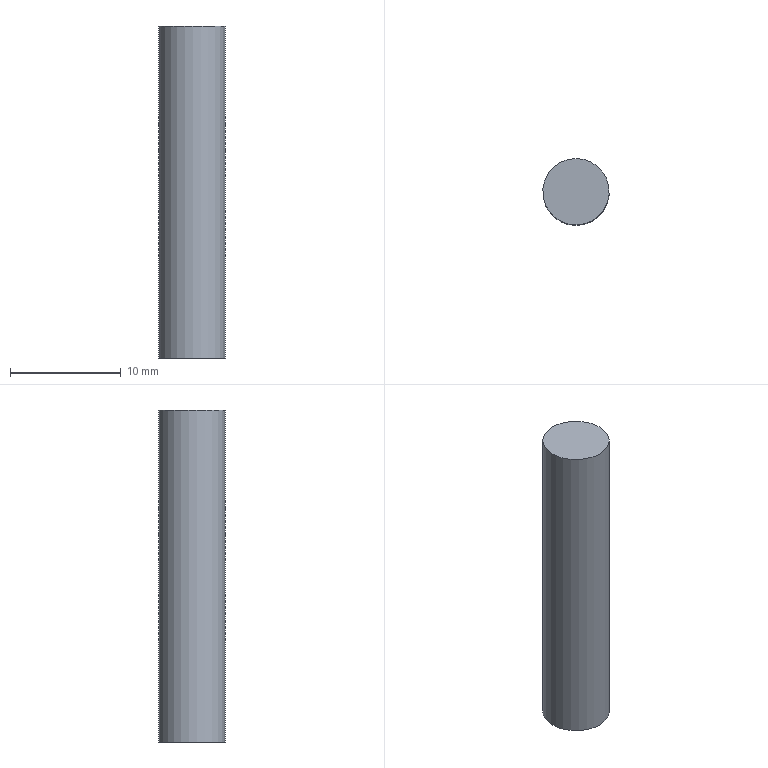Component | NX | PIN_A6X30_2 | 1 solid | 3 faces | box 6 x 6 x 30 mm | volume 848 mm3 | plane 2 | cylinder 1 | commonest cylinder face diameters 6 x1
STEP:
#1=CARTESIAN_POINT('',(0.,0.,0.));
#2=DIRECTION('',(0.,0.,1.));
#3=DIRECTION('',(1.,0.,0.));
#4=AXIS2_PLACEMENT_3D('',#1,#2,#3);
#5=CARTESIAN_POINT('',(56.729,7.851,-9.));
#6=VERTEX_POINT('',#5);
#7=CARTESIAN_POINT('',(59.5,9.,-9.));
#8=DIRECTION('',(0.,0.,1.));
#9=DIRECTION('',(-0.9237,-0.383,0.));
#10=AXIS2_PLACEMENT_3D('',#7,#8,#9);
#11=CIRCLE('',#10,3.);
#12=CARTESIAN_POINT('',(59.5,9.,-9.));
#13=DIRECTION('',(0.,0.,-1.));
#14=DIRECTION('',(-0.9237,-0.383,0.));
#15=AXIS2_PLACEMENT_3D('',#12,#13,#14);
#16=PLANE('',#15);
#17=CARTESIAN_POINT('',(3.,0.));
#18=CARTESIAN_POINT('',(3.,-5.196));
#19=CARTESIAN_POINT('',(-1.5,-2.598));
#20=CARTESIAN_POINT('',(-6.,-0.));
#21=CARTESIAN_POINT('',(-1.5,2.598));
#22=CARTESIAN_POINT('',(3.,5.196));
#23=CARTESIAN_POINT('',(3.,0.));
#24=(BOUNDED_CURVE()B_SPLINE_CURVE(2,(#17,#18,#19,#20,#21,#22,#23),.UNSPECIFIED.,.T.,.F.)B_SPLINE_CURVE_WITH_KNOTS((1,2,2,2,2,1),(-2.094,0.,2.094,4.189,6.283,8.378),.UNSPECIFIED.)CURVE()GEOMETRIC_REPRESENTATION_ITEM()RATIONAL_B_SPLINE_CURVE((1.,0.5,1.,0.5,1.,0.5,1.))REPRESENTATION_ITEM(''));
#25=(GEOMETRIC_REPRESENTATION_CONTEXT(2)PARAMETRIC_REPRESENTATION_CONTEXT()REPRESENTATION_CONTEXT('',''));
#26=DEFINITIONAL_REPRESENTATION('',(#24),#25);
#27=PCURVE('',#16,#26);
#28=CARTESIAN_POINT('',(59.5,9.,21.));
#29=DIRECTION('',(0.,0.,-1.));
#30=DIRECTION('',(-0.9237,-0.383,0.));
#31=AXIS2_PLACEMENT_3D('',#28,#29,#30);
#32=CYLINDRICAL_SURFACE('',#31,3.);
#33=CARTESIAN_POINT('',(6.283,30.));
#34=DIRECTION('',(-1.,0.));
#35=VECTOR('',#34,1.);
#36=LINE('',#33,#35);
#37=(GEOMETRIC_REPRESENTATION_CONTEXT(2)PARAMETRIC_REPRESENTATION_CONTEXT()REPRESENTATION_CONTEXT('',''));
#38=DEFINITIONAL_REPRESENTATION('',(#36),#37);
#39=PCURVE('',#32,#38);
#40=SURFACE_CURVE('',#11,(#27,#39),.PCURVE_S1.);
#41=EDGE_CURVE('',#6,#6,#40,.T.);
#42=ORIENTED_EDGE('',*,*,#41,.F.);
#43=EDGE_LOOP('',(#42));
#44=FACE_BOUND('',#43,.T.);
#45=ADVANCED_FACE('',(#44),#16,.T.);
#46=CARTESIAN_POINT('',(56.729,7.851,21.));
#47=VERTEX_POINT('',#46);
#48=CARTESIAN_POINT('',(59.5,9.,21.));
#49=DIRECTION('',(0.,0.,-1.));
#50=DIRECTION('',(-0.9237,-0.383,0.));
#51=AXIS2_PLACEMENT_3D('',#48,#49,#50);
#52=CIRCLE('',#51,3.);
#53=CARTESIAN_POINT('',(59.5,9.,21.));
#54=DIRECTION('',(0.,0.,1.));
#55=DIRECTION('',(0.9237,0.383,0.));
#56=AXIS2_PLACEMENT_3D('',#53,#54,#55);
#57=PLANE('',#56);
#58=CARTESIAN_POINT('',(-3.,0.));
#59=CARTESIAN_POINT('',(-3.,5.196));
#60=CARTESIAN_POINT('',(1.5,2.598));
#61=CARTESIAN_POINT('',(6.,-0.));
#62=CARTESIAN_POINT('',(1.5,-2.598));
#63=CARTESIAN_POINT('',(-3.,-5.196));
#64=CARTESIAN_POINT('',(-3.,0.));
#65=(BOUNDED_CURVE()B_SPLINE_CURVE(2,(#58,#59,#60,#61,#62,#63,#64),.UNSPECIFIED.,.T.,.F.)B_SPLINE_CURVE_WITH_KNOTS((1,2,2,2,2,1),(-2.094,0.,2.094,4.189,6.283,8.378),.UNSPECIFIED.)CURVE()GEOMETRIC_REPRESENTATION_ITEM()RATIONAL_B_SPLINE_CURVE((1.,0.5,1.,0.5,1.,0.5,1.))REPRESENTATION_ITEM(''));
#66=(GEOMETRIC_REPRESENTATION_CONTEXT(2)PARAMETRIC_REPRESENTATION_CONTEXT()REPRESENTATION_CONTEXT('',''));
#67=DEFINITIONAL_REPRESENTATION('',(#65),#66);
#68=PCURVE('',#57,#67);
#69=CARTESIAN_POINT('',(0.,0.));
#70=DIRECTION('',(1.,0.));
#71=VECTOR('',#70,1.);
#72=LINE('',#69,#71);
#73=(GEOMETRIC_REPRESENTATION_CONTEXT(2)PARAMETRIC_REPRESENTATION_CONTEXT()REPRESENTATION_CONTEXT('',''));
#74=DEFINITIONAL_REPRESENTATION('',(#72),#73);
#75=PCURVE('',#32,#74);
#76=SURFACE_CURVE('',#52,(#68,#75),.PCURVE_S1.);
#77=EDGE_CURVE('',#47,#47,#76,.T.);
#78=ORIENTED_EDGE('',*,*,#77,.F.);
#79=EDGE_LOOP('',(#78));
#80=FACE_BOUND('',#79,.T.);
#81=ADVANCED_FACE('',(#80),#57,.T.);
#82=ORIENTED_EDGE('',*,*,#41,.T.);
#83=CARTESIAN_POINT('',(56.729,7.851,21.));
#84=CARTESIAN_POINT('',(56.729,7.851,-9.));
#85=B_SPLINE_CURVE_WITH_KNOTS('',1,(#83,#84),.UNSPECIFIED.,.F.,.F.,(2,2),(0.,30.),.PIECEWISE_BEZIER_KNOTS.);
#86=CARTESIAN_POINT('',(0.,0.));
#87=DIRECTION('',(0.,1.));
#88=VECTOR('',#87,1.);
#89=LINE('',#86,#88);
#90=(GEOMETRIC_REPRESENTATION_CONTEXT(2)PARAMETRIC_REPRESENTATION_CONTEXT()REPRESENTATION_CONTEXT('',''));
#91=DEFINITIONAL_REPRESENTATION('',(#89),#90);
#92=PCURVE('',#32,#91);
#93=CARTESIAN_POINT('',(6.283,0.));
#94=DIRECTION('',(0.,1.));
#95=VECTOR('',#94,1.);
#96=LINE('',#93,#95);
#97=(GEOMETRIC_REPRESENTATION_CONTEXT(2)PARAMETRIC_REPRESENTATION_CONTEXT()REPRESENTATION_CONTEXT('',''));
#98=DEFINITIONAL_REPRESENTATION('',(#96),#97);
#99=PCURVE('',#32,#98);
#100=SEAM_CURVE('',#85,(#92,#99),.PCURVE_S1.);
#101=EDGE_CURVE('',#47,#6,#100,.T.);
#102=ORIENTED_EDGE('',*,*,#101,.F.);
#103=ORIENTED_EDGE('',*,*,#77,.T.);
#104=ORIENTED_EDGE('',*,*,#101,.T.);
#105=EDGE_LOOP('',(#82,#102,#103,#104));
#106=FACE_BOUND('',#105,.T.);
#107=ADVANCED_FACE('',(#106),#32,.T.);
#108=CLOSED_SHELL('',(#45,#81,#107));
#109=MANIFOLD_SOLID_BREP('',#108);
#110=(LENGTH_UNIT()NAMED_UNIT(*)SI_UNIT(.MILLI.,.METRE.));
#111=UNCERTAINTY_MEASURE_WITH_UNIT(LENGTH_MEASURE(0.00001),#110,'','');
#112=(NAMED_UNIT(*)PLANE_ANGLE_UNIT()SI_UNIT($,.RADIAN.));
#113=(NAMED_UNIT(*)SI_UNIT($,.STERADIAN.)SOLID_ANGLE_UNIT());
#114=(GEOMETRIC_REPRESENTATION_CONTEXT(3)GLOBAL_UNCERTAINTY_ASSIGNED_CONTEXT((#111))GLOBAL_UNIT_ASSIGNED_CONTEXT((#110,#112,#113))REPRESENTATION_CONTEXT('',''));
#115=ADVANCED_BREP_SHAPE_REPRESENTATION('',(#4,#109),#114);